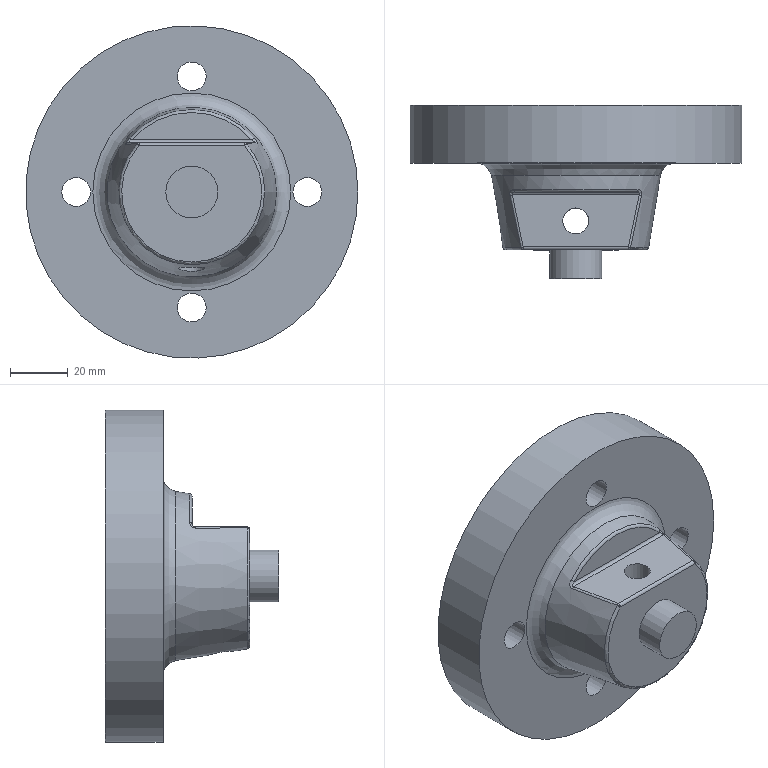Component | NX | BASE | 1 solid | 25 faces | volume 268022 mm3 | cylinder 9 | plane 6 | spline 4 | torus 3 | sphere 2 | cone 1 | commonest cylinder face diameters 10 x4 2 x2 115 x1 18 x1 9 x1